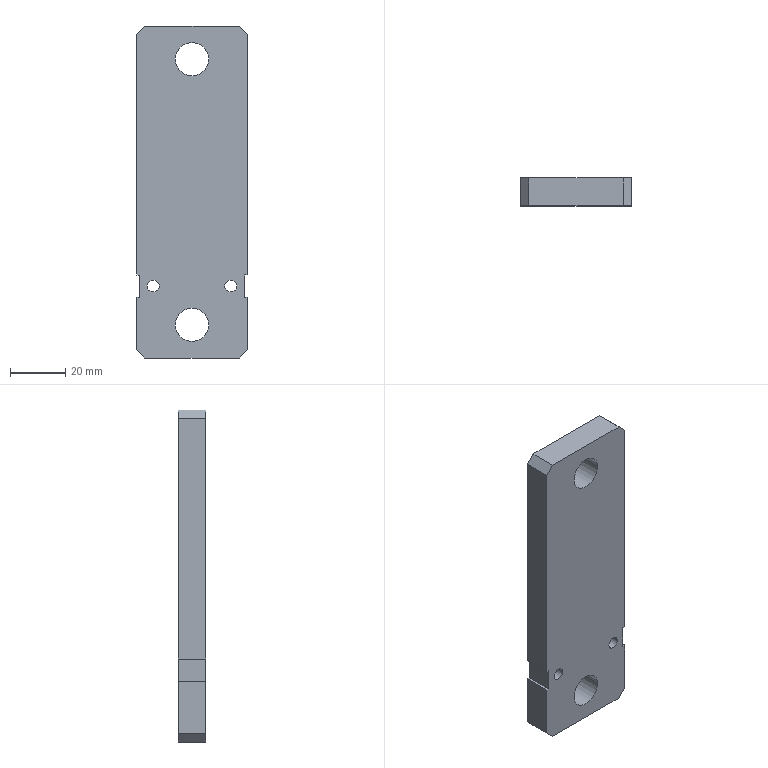Component | SolidWorks | HandlingMechanism-2_A071-1 | 1 solid | 32 faces | box 40 x 10 x 120 mm | volume 44793 mm3 | plane 20 | cylinder 12 | commonest cylinder face diameters 8 x4 4.3 x4 12 x4
build123d program:
from build123d import *

# Parameters (mm, degrees)
SKETCH4_W                                       = 40
SKETCH4_H                                       = 120
BOSS_EXTRUDE3_DEPTH                             = 10
CHAMFER1_SIZE                                   = 3
M12X1_TAPPED_HOLE1_D                            = 12
M12X1_TAPPED_HOLE1_DEPTH                        = 26.25
M12X1_TAPPED_HOLE1_TIP                          = 3.605
SKETCH8_W                                       = 1
SKETCH8_H                                       = 8
CUT_EXTRUDE2_DEPTH                              = 20
M4_HEX_SOCKET_HEAD_CAP_SCREW_CBORE1_D           = 4.3
M4_HEX_SOCKET_HEAD_CAP_SCREW_CBORE1_CBORE_D     = 8
M4_HEX_SOCKET_HEAD_CAP_SCREW_CBORE1_CBORE_DEPTH = 4.4


with BuildPart() as part:
    # Sketch4 → Boss-Extrude3 (new body)
    with BuildSketch(Plane(origin=(0, 0, 0), x_dir=(-1, 0, 0), z_dir=(0, 0, -1))):
        Rectangle(SKETCH4_W, SKETCH4_H)
    extrude(amount=BOSS_EXTRUDE3_DEPTH)

    # Chamfer1
    chamfer1_edges = [part.edges().sort_by_distance(p)[0] for p in [
        (20, 60, -5),
        (-20, 60, -5),
        (-20, -60, -5),
        (20, -60, -5),
    ]]
    chamfer(chamfer1_edges, length=CHAMFER1_SIZE)

    # M12x1 Tapped Hole1
    with Locations(Plane(origin=(0, 0, -10), x_dir=(-1, 0, 0), z_dir=(0, 0, -1))):
        with Locations((0, -48), (0, 48)):
            Hole(M12X1_TAPPED_HOLE1_D / 2, depth=M12X1_TAPPED_HOLE1_DEPTH)
            with Locations((0, 0, -(M12X1_TAPPED_HOLE1_DEPTH + M12X1_TAPPED_HOLE1_TIP / 2))):  # 118° drill point
                Cone(0, M12X1_TAPPED_HOLE1_D / 2, M12X1_TAPPED_HOLE1_TIP, mode=Mode.SUBTRACT)

    # Sketch8 → Cut-Extrude2 (cut)
    with BuildSketch(Plane(origin=(0, 0, -10), x_dir=(-1, 0, 0), z_dir=(0, 0, -1))):
        with Locations((19.5, 34)):
            Rectangle(SKETCH8_W, SKETCH8_H)
        with Locations((-19.5, 34)):
            Rectangle(SKETCH8_W, SKETCH8_H)
    extrude(amount=-CUT_EXTRUDE2_DEPTH, mode=Mode.SUBTRACT)

    # M4 Hex Socket Head Cap Screw CBORE1 (through all)
    with Locations(Plane(origin=(0, 0, -10), x_dir=(-1, 0, 0), z_dir=(0, 0, -1))):
        with Locations((-14, 34), (14, 34)):
            CounterBoreHole(M4_HEX_SOCKET_HEAD_CAP_SCREW_CBORE1_D / 2, M4_HEX_SOCKET_HEAD_CAP_SCREW_CBORE1_CBORE_D / 2, M4_HEX_SOCKET_HEAD_CAP_SCREW_CBORE1_CBORE_DEPTH)


solid = part.part

# Placed as in the assembly
solid = solid.moved(Location((25.881, 208.5, 187), (90, 0, -180)))
STEP:
#1=COLOUR_RGB('',0.7922,0.8196,0.9333);
#2=FILL_AREA_STYLE_COLOUR('',#1);
#3=FILL_AREA_STYLE('',(#2));
#4=SURFACE_STYLE_FILL_AREA(#3);
#5=SURFACE_SIDE_STYLE('',(#4));
#6=SURFACE_STYLE_USAGE(.BOTH.,#5);
#7=PRESENTATION_STYLE_ASSIGNMENT((#6));
#8=CARTESIAN_POINT('',(0.3103,8.429,6.024));
#9=VERTEX_POINT('',#8);
#10=CARTESIAN_POINT('',(0.6252,8.429,6.024));
#11=VERTEX_POINT('',#10);
#12=CARTESIAN_POINT('',(0.4677,8.429,6.024));
#13=DIRECTION('',(0.,1.,-0.));
#14=DIRECTION('',(1.,0.,0.));
#15=AXIS2_PLACEMENT_3D('',#12,#13,#14);
#16=CIRCLE('',#15,0.1575);
#17=EDGE_CURVE('',#9,#11,#16,.T.);
#18=ORIENTED_EDGE('',*,*,#17,.F.);
#19=CARTESIAN_POINT('',(0.3103,8.602,6.024));
#20=VERTEX_POINT('',#19);
#21=CARTESIAN_POINT('',(0.3103,8.602,6.024));
#22=DIRECTION('',(0.,1.,-0.));
#23=VECTOR('',#22,39.37);
#24=LINE('',#21,#23);
#25=EDGE_CURVE('',#9,#20,#24,.T.);
#26=ORIENTED_EDGE('',*,*,#25,.T.);
#27=CARTESIAN_POINT('',(0.6252,8.602,6.024));
#28=VERTEX_POINT('',#27);
#29=CARTESIAN_POINT('',(0.4677,8.602,6.024));
#30=DIRECTION('',(0.,1.,-0.));
#31=DIRECTION('',(1.,0.,0.));
#32=AXIS2_PLACEMENT_3D('',#29,#30,#31);
#33=CIRCLE('',#32,0.1575);
#34=EDGE_CURVE('',#20,#28,#33,.T.);
#35=ORIENTED_EDGE('',*,*,#34,.T.);
#36=CARTESIAN_POINT('',(0.6252,8.602,6.024));
#37=DIRECTION('',(0.,1.,-0.));
#38=VECTOR('',#37,39.37);
#39=LINE('',#36,#38);
#40=EDGE_CURVE('',#11,#28,#39,.T.);
#41=ORIENTED_EDGE('',*,*,#40,.F.);
#42=EDGE_LOOP('',(#18,#26,#35,#41));
#43=FACE_OUTER_BOUND('',#42,.T.);
#44=CARTESIAN_POINT('',(0.4677,8.602,6.024));
#45=DIRECTION('',(0.,1.,-0.));
#46=DIRECTION('',(1.,0.,0.));
#47=AXIS2_PLACEMENT_3D('',#44,#45,#46);
#48=CYLINDRICAL_SURFACE('',#47,0.1575);
#49=ADVANCED_FACE('',(#43),#48,.F.);
#50=CARTESIAN_POINT('',(0.3831,8.209,6.024));
#51=VERTEX_POINT('',#50);
#52=CARTESIAN_POINT('',(0.5524,8.209,6.024));
#53=VERTEX_POINT('',#52);
#54=CARTESIAN_POINT('',(0.4677,8.209,6.024));
#55=DIRECTION('',(0.,1.,-0.));
#56=DIRECTION('',(1.,0.,0.));
#57=AXIS2_PLACEMENT_3D('',#54,#55,#56);
#58=CIRCLE('',#57,0.08465);
#59=EDGE_CURVE('',#51,#53,#58,.T.);
#60=ORIENTED_EDGE('',*,*,#59,.F.);
#61=CARTESIAN_POINT('',(0.3831,8.429,6.024));
#62=VERTEX_POINT('',#61);
#63=CARTESIAN_POINT('',(0.3831,8.602,6.024));
#64=DIRECTION('',(0.,1.,-0.));
#65=VECTOR('',#64,39.37);
#66=LINE('',#63,#65);
#67=EDGE_CURVE('',#51,#62,#66,.T.);
#68=ORIENTED_EDGE('',*,*,#67,.T.);
#69=CARTESIAN_POINT('',(0.5524,8.429,6.024));
#70=VERTEX_POINT('',#69);
#71=CARTESIAN_POINT('',(0.4677,8.429,6.024));
#72=DIRECTION('',(0.,1.,-0.));
#73=DIRECTION('',(1.,0.,0.));
#74=AXIS2_PLACEMENT_3D('',#71,#72,#73);
#75=CIRCLE('',#74,0.08465);
#76=EDGE_CURVE('',#62,#70,#75,.T.);
#77=ORIENTED_EDGE('',*,*,#76,.T.);
#78=CARTESIAN_POINT('',(0.5524,8.602,6.024));
#79=DIRECTION('',(0.,1.,-0.));
#80=VECTOR('',#79,39.37);
#81=LINE('',#78,#80);
#82=EDGE_CURVE('',#53,#70,#81,.T.);
#83=ORIENTED_EDGE('',*,*,#82,.F.);
#84=EDGE_LOOP('',(#60,#68,#77,#83));
#85=FACE_OUTER_BOUND('',#84,.T.);
#86=CARTESIAN_POINT('',(0.4677,8.602,6.024));
#87=DIRECTION('',(0.,1.,-0.));
#88=DIRECTION('',(1.,0.,0.));
#89=AXIS2_PLACEMENT_3D('',#86,#87,#88);
#90=CYLINDRICAL_SURFACE('',#89,0.08465);
#91=ADVANCED_FACE('',(#85),#90,.F.);
#92=CARTESIAN_POINT('',(1.413,8.429,6.024));
#93=VERTEX_POINT('',#92);
#94=CARTESIAN_POINT('',(1.728,8.429,6.024));
#95=VERTEX_POINT('',#94);
#96=CARTESIAN_POINT('',(1.57,8.429,6.024));
#97=DIRECTION('',(0.,1.,-0.));
#98=DIRECTION('',(1.,0.,0.));
#99=AXIS2_PLACEMENT_3D('',#96,#97,#98);
#100=CIRCLE('',#99,0.1575);
#101=EDGE_CURVE('',#93,#95,#100,.T.);
#102=ORIENTED_EDGE('',*,*,#101,.F.);
#103=CARTESIAN_POINT('',(1.413,8.602,6.024));
#104=VERTEX_POINT('',#103);
#105=CARTESIAN_POINT('',(1.413,8.602,6.024));
#106=DIRECTION('',(0.,1.,-0.));
#107=VECTOR('',#106,39.37);
#108=LINE('',#105,#107);
#109=EDGE_CURVE('',#93,#104,#108,.T.);
#110=ORIENTED_EDGE('',*,*,#109,.T.);
#111=CARTESIAN_POINT('',(1.728,8.602,6.024));
#112=VERTEX_POINT('',#111);
#113=CARTESIAN_POINT('',(1.57,8.602,6.024));
#114=DIRECTION('',(0.,1.,-0.));
#115=DIRECTION('',(1.,0.,0.));
#116=AXIS2_PLACEMENT_3D('',#113,#114,#115);
#117=CIRCLE('',#116,0.1575);
#118=EDGE_CURVE('',#104,#112,#117,.T.);
#119=ORIENTED_EDGE('',*,*,#118,.T.);
#120=CARTESIAN_POINT('',(1.728,8.602,6.024));
#121=DIRECTION('',(0.,1.,-0.));
#122=VECTOR('',#121,39.37);
#123=LINE('',#120,#122);
#124=EDGE_CURVE('',#95,#112,#123,.T.);
#125=ORIENTED_EDGE('',*,*,#124,.F.);
#126=EDGE_LOOP('',(#102,#110,#119,#125));
#127=FACE_OUTER_BOUND('',#126,.T.);
#128=CARTESIAN_POINT('',(1.57,8.602,6.024));
#129=DIRECTION('',(0.,1.,-0.));
#130=DIRECTION('',(1.,0.,0.));
#131=AXIS2_PLACEMENT_3D('',#128,#129,#130);
#132=CYLINDRICAL_SURFACE('',#131,0.1575);
#133=ADVANCED_FACE('',(#127),#132,.F.);
#134=CARTESIAN_POINT('',(1.485,8.209,6.024));
#135=VERTEX_POINT('',#134);
#136=CARTESIAN_POINT('',(1.655,8.209,6.024));
#137=VERTEX_POINT('',#136);
#138=CARTESIAN_POINT('',(1.57,8.209,6.024));
#139=DIRECTION('',(0.,1.,-0.));
#140=DIRECTION('',(1.,0.,0.));
#141=AXIS2_PLACEMENT_3D('',#138,#139,#140);
#142=CIRCLE('',#141,0.08465);
#143=EDGE_CURVE('',#135,#137,#142,.T.);
#144=ORIENTED_EDGE('',*,*,#143,.F.);
#145=CARTESIAN_POINT('',(1.485,8.429,6.024));
#146=VERTEX_POINT('',#145);
#147=CARTESIAN_POINT('',(1.485,8.602,6.024));
#148=DIRECTION('',(0.,1.,-0.));
#149=VECTOR('',#148,39.37);
#150=LINE('',#147,#149);
#151=EDGE_CURVE('',#135,#146,#150,.T.);
#152=ORIENTED_EDGE('',*,*,#151,.T.);
#153=CARTESIAN_POINT('',(1.655,8.429,6.024));
#154=VERTEX_POINT('',#153);
#155=CARTESIAN_POINT('',(1.57,8.429,6.024));
#156=DIRECTION('',(0.,1.,-0.));
#157=DIRECTION('',(1.,0.,0.));
#158=AXIS2_PLACEMENT_3D('',#155,#156,#157);
#159=CIRCLE('',#158,0.08465);
#160=EDGE_CURVE('',#146,#154,#159,.T.);
#161=ORIENTED_EDGE('',*,*,#160,.T.);
#162=CARTESIAN_POINT('',(1.655,8.602,6.024));
#163=DIRECTION('',(0.,1.,-0.));
#164=VECTOR('',#163,39.37);
#165=LINE('',#162,#164);
#166=EDGE_CURVE('',#137,#154,#165,.T.);
#167=ORIENTED_EDGE('',*,*,#166,.F.);
#168=EDGE_LOOP('',(#144,#152,#161,#167));
#169=FACE_OUTER_BOUND('',#168,.T.);
#170=CARTESIAN_POINT('',(1.57,8.602,6.024));
#171=DIRECTION('',(0.,1.,-0.));
#172=DIRECTION('',(1.,0.,0.));
#173=AXIS2_PLACEMENT_3D('',#170,#171,#172);
#174=CYLINDRICAL_SURFACE('',#173,0.08465);
#175=ADVANCED_FACE('',(#169),#174,.F.);
#176=CARTESIAN_POINT('',(1.255,8.209,9.252));
#177=VERTEX_POINT('',#176);
#178=CARTESIAN_POINT('',(0.7827,8.209,9.252));
#179=VERTEX_POINT('',#178);
#180=CARTESIAN_POINT('',(1.019,8.209,9.252));
#181=DIRECTION('',(-0.,-1.,0.));
#182=DIRECTION('',(-1.,0.,0.));
#183=AXIS2_PLACEMENT_3D('',#180,#181,#182);
#184=CIRCLE('',#183,0.2362);
#185=EDGE_CURVE('',#177,#179,#184,.T.);
#186=ORIENTED_EDGE('',*,*,#185,.T.);
#187=CARTESIAN_POINT('',(0.7827,8.602,9.252));
#188=VERTEX_POINT('',#187);
#189=CARTESIAN_POINT('',(0.7827,8.602,9.252));
#190=DIRECTION('',(0.,1.,-0.));
#191=VECTOR('',#190,39.37);
#192=LINE('',#189,#191);
#193=EDGE_CURVE('',#179,#188,#192,.T.);
#194=ORIENTED_EDGE('',*,*,#193,.T.);
#195=CARTESIAN_POINT('',(1.255,8.602,9.252));
#196=VERTEX_POINT('',#195);
#197=CARTESIAN_POINT('',(1.019,8.602,9.252));
#198=DIRECTION('',(0.,1.,-0.));
#199=DIRECTION('',(1.,0.,0.));
#200=AXIS2_PLACEMENT_3D('',#197,#198,#199);
#201=CIRCLE('',#200,0.2362);
#202=EDGE_CURVE('',#188,#196,#201,.T.);
#203=ORIENTED_EDGE('',*,*,#202,.T.);
#204=CARTESIAN_POINT('',(1.255,8.602,9.252));
#205=DIRECTION('',(0.,1.,-0.));
#206=VECTOR('',#205,39.37);
#207=LINE('',#204,#206);
#208=EDGE_CURVE('',#177,#196,#207,.T.);
#209=ORIENTED_EDGE('',*,*,#208,.F.);
#210=EDGE_LOOP('',(#186,#194,#203,#209));
#211=FACE_OUTER_BOUND('',#210,.T.);
#212=CARTESIAN_POINT('',(1.019,8.602,9.252));
#213=DIRECTION('',(0.,1.,-0.));
#214=DIRECTION('',(1.,0.,0.));
#215=AXIS2_PLACEMENT_3D('',#212,#213,#214);
#216=CYLINDRICAL_SURFACE('',#215,0.2362);
#217=ADVANCED_FACE('',(#211),#216,.F.);
#218=CARTESIAN_POINT('',(1.255,8.209,5.472));
#219=VERTEX_POINT('',#218);
#220=CARTESIAN_POINT('',(0.7827,8.209,5.472));
#221=VERTEX_POINT('',#220);
#222=CARTESIAN_POINT('',(1.019,8.209,5.472));
#223=DIRECTION('',(-0.,-1.,0.));
#224=DIRECTION('',(-1.,0.,0.));
#225=AXIS2_PLACEMENT_3D('',#222,#223,#224);
#226=CIRCLE('',#225,0.2362);
#227=EDGE_CURVE('',#219,#221,#226,.T.);
#228=ORIENTED_EDGE('',*,*,#227,.T.);
#229=CARTESIAN_POINT('',(0.7827,8.602,5.472));
#230=VERTEX_POINT('',#229);
#231=CARTESIAN_POINT('',(0.7827,8.602,5.472));
#232=DIRECTION('',(0.,1.,-0.));
#233=VECTOR('',#232,39.37);
#234=LINE('',#231,#233);
#235=EDGE_CURVE('',#221,#230,#234,.T.);
#236=ORIENTED_EDGE('',*,*,#235,.T.);
#237=CARTESIAN_POINT('',(1.255,8.602,5.472));
#238=VERTEX_POINT('',#237);
#239=CARTESIAN_POINT('',(1.019,8.602,5.472));
#240=DIRECTION('',(0.,1.,-0.));
#241=DIRECTION('',(1.,0.,0.));
#242=AXIS2_PLACEMENT_3D('',#239,#240,#241);
#243=CIRCLE('',#242,0.2362);
#244=EDGE_CURVE('',#230,#238,#243,.T.);
#245=ORIENTED_EDGE('',*,*,#244,.T.);
#246=CARTESIAN_POINT('',(1.255,8.602,5.472));
#247=DIRECTION('',(0.,1.,-0.));
#248=VECTOR('',#247,39.37);
#249=LINE('',#246,#248);
#250=EDGE_CURVE('',#219,#238,#249,.T.);
#251=ORIENTED_EDGE('',*,*,#250,.F.);
#252=EDGE_LOOP('',(#228,#236,#245,#251));
#253=FACE_OUTER_BOUND('',#252,.T.);
#254=CARTESIAN_POINT('',(1.019,8.602,5.472));
#255=DIRECTION('',(0.,1.,-0.));
#256=DIRECTION('',(1.,0.,0.));
#257=AXIS2_PLACEMENT_3D('',#254,#255,#256);
#258=CYLINDRICAL_SURFACE('',#257,0.2362);
#259=ADVANCED_FACE('',(#253),#258,.F.);
#260=CARTESIAN_POINT('',(1.57,8.602,6.024));
#261=DIRECTION('',(0.,1.,-0.));
#262=DIRECTION('',(1.,0.,0.));
#263=AXIS2_PLACEMENT_3D('',#260,#261,#262);
#264=CIRCLE('',#263,0.1575);
#265=EDGE_CURVE('',#112,#104,#264,.T.);
#266=ORIENTED_EDGE('',*,*,#265,.F.);
#267=ORIENTED_EDGE('',*,*,#118,.F.);
#268=EDGE_LOOP('',(#266,#267));
#269=FACE_BOUND('',#268,.T.);
#270=CARTESIAN_POINT('',(1.019,8.602,9.252));
#271=DIRECTION('',(0.,1.,-0.));
#272=DIRECTION('',(1.,0.,0.));
#273=AXIS2_PLACEMENT_3D('',#270,#271,#272);
#274=CIRCLE('',#273,0.2362);
#275=EDGE_CURVE('',#196,#188,#274,.T.);
#276=ORIENTED_EDGE('',*,*,#275,.F.);
#277=ORIENTED_EDGE('',*,*,#202,.F.);
#278=EDGE_LOOP('',(#276,#277));
#279=FACE_BOUND('',#278,.T.);
#280=CARTESIAN_POINT('',(1.019,8.602,5.472));
#281=DIRECTION('',(0.,1.,-0.));
#282=DIRECTION('',(1.,0.,0.));
#283=AXIS2_PLACEMENT_3D('',#280,#281,#282);
#284=CIRCLE('',#283,0.2362);
#285=EDGE_CURVE('',#238,#230,#284,.T.);
#286=ORIENTED_EDGE('',*,*,#285,.F.);
#287=ORIENTED_EDGE('',*,*,#244,.F.);
#288=EDGE_LOOP('',(#286,#287));
#289=FACE_BOUND('',#288,.T.);
#290=CARTESIAN_POINT('',(0.2709,8.602,6.181));
#291=VERTEX_POINT('',#290);
#292=CARTESIAN_POINT('',(0.2709,8.602,5.866));
#293=VERTEX_POINT('',#292);
#294=CARTESIAN_POINT('',(0.2709,8.602,5.866));
#295=DIRECTION('',(0.,-0.,-1.));
#296=VECTOR('',#295,39.37);
#297=LINE('',#294,#296);
#298=EDGE_CURVE('',#291,#293,#297,.T.);
#299=ORIENTED_EDGE('',*,*,#298,.F.);
#300=CARTESIAN_POINT('',(0.2315,8.602,6.181));
#301=VERTEX_POINT('',#300);
#302=CARTESIAN_POINT('',(0.2709,8.602,6.181));
#303=DIRECTION('',(1.,-0.,0.));
#304=VECTOR('',#303,39.37);
#305=LINE('',#302,#304);
#306=EDGE_CURVE('',#301,#291,#305,.T.);
#307=ORIENTED_EDGE('',*,*,#306,.F.);
#308=CARTESIAN_POINT('',(0.2315,8.602,9.606));
#309=VERTEX_POINT('',#308);
#310=CARTESIAN_POINT('',(0.2315,8.602,9.724));
#311=DIRECTION('',(-0.,0.,1.));
#312=VECTOR('',#311,39.37);
#313=LINE('',#310,#312);
#314=EDGE_CURVE('',#301,#309,#313,.T.);
#315=ORIENTED_EDGE('',*,*,#314,.T.);
#316=CARTESIAN_POINT('',(0.3496,8.602,9.724));
#317=VERTEX_POINT('',#316);
#318=CARTESIAN_POINT('',(0.3496,8.602,9.724));
#319=DIRECTION('',(0.7071,-0.,0.7071));
#320=VECTOR('',#319,39.37);
#321=LINE('',#318,#320);
#322=EDGE_CURVE('',#309,#317,#321,.T.);
#323=ORIENTED_EDGE('',*,*,#322,.T.);
#324=CARTESIAN_POINT('',(1.688,8.602,9.724));
#325=VERTEX_POINT('',#324);
#326=CARTESIAN_POINT('',(0.2315,8.602,9.724));
#327=DIRECTION('',(1.,-0.,0.));
#328=VECTOR('',#327,39.37);
#329=LINE('',#326,#328);
#330=EDGE_CURVE('',#317,#325,#329,.T.);
#331=ORIENTED_EDGE('',*,*,#330,.T.);
#332=CARTESIAN_POINT('',(1.806,8.602,9.606));
#333=VERTEX_POINT('',#332);
#334=CARTESIAN_POINT('',(1.806,8.602,9.606));
#335=DIRECTION('',(0.7071,-0.,-0.7071));
#336=VECTOR('',#335,39.37);
#337=LINE('',#334,#336);
#338=EDGE_CURVE('',#325,#333,#337,.T.);
#339=ORIENTED_EDGE('',*,*,#338,.T.);
#340=CARTESIAN_POINT('',(1.806,8.602,6.181));
#341=VERTEX_POINT('',#340);
#342=CARTESIAN_POINT('',(1.806,8.602,9.724));
#343=DIRECTION('',(0.,-0.,-1.));
#344=VECTOR('',#343,39.37);
#345=LINE('',#342,#344);
#346=EDGE_CURVE('',#333,#341,#345,.T.);
#347=ORIENTED_EDGE('',*,*,#346,.T.);
#348=CARTESIAN_POINT('',(1.767,8.602,6.181));
#349=VERTEX_POINT('',#348);
#350=CARTESIAN_POINT('',(1.767,8.602,6.181));
#351=DIRECTION('',(1.,-0.,0.));
#352=VECTOR('',#351,39.37);
#353=LINE('',#350,#352);
#354=EDGE_CURVE('',#349,#341,#353,.T.);
#355=ORIENTED_EDGE('',*,*,#354,.F.);
#356=CARTESIAN_POINT('',(1.767,8.602,5.866));
#357=VERTEX_POINT('',#356);
#358=CARTESIAN_POINT('',(1.767,8.602,5.866));
#359=DIRECTION('',(-0.,0.,1.));
#360=VECTOR('',#359,39.37);
#361=LINE('',#358,#360);
#362=EDGE_CURVE('',#357,#349,#361,.T.);
#363=ORIENTED_EDGE('',*,*,#362,.F.);
#364=CARTESIAN_POINT('',(1.806,8.602,5.866));
#365=VERTEX_POINT('',#364);
#366=CARTESIAN_POINT('',(1.767,8.602,5.866));
#367=DIRECTION('',(-1.,0.,-0.));
#368=VECTOR('',#367,39.37);
#369=LINE('',#366,#368);
#370=EDGE_CURVE('',#365,#357,#369,.T.);
#371=ORIENTED_EDGE('',*,*,#370,.F.);
#372=CARTESIAN_POINT('',(1.806,8.602,5.118));
#373=VERTEX_POINT('',#372);
#374=CARTESIAN_POINT('',(1.806,8.602,9.724));
#375=DIRECTION('',(0.,-0.,-1.));
#376=VECTOR('',#375,39.37);
#377=LINE('',#374,#376);
#378=EDGE_CURVE('',#365,#373,#377,.T.);
#379=ORIENTED_EDGE('',*,*,#378,.T.);
#380=CARTESIAN_POINT('',(1.688,8.602,5.));
#381=VERTEX_POINT('',#380);
#382=CARTESIAN_POINT('',(1.688,8.602,5.));
#383=DIRECTION('',(-0.7071,0.,-0.7071));
#384=VECTOR('',#383,39.37);
#385=LINE('',#382,#384);
#386=EDGE_CURVE('',#373,#381,#385,.T.);
#387=ORIENTED_EDGE('',*,*,#386,.T.);
#388=CARTESIAN_POINT('',(0.3496,8.602,5.));
#389=VERTEX_POINT('',#388);
#390=CARTESIAN_POINT('',(0.2315,8.602,5.));
#391=DIRECTION('',(-1.,0.,-0.));
#392=VECTOR('',#391,39.37);
#393=LINE('',#390,#392);
#394=EDGE_CURVE('',#381,#389,#393,.T.);
#395=ORIENTED_EDGE('',*,*,#394,.T.);
#396=CARTESIAN_POINT('',(0.2315,8.602,5.118));
#397=VERTEX_POINT('',#396);
#398=CARTESIAN_POINT('',(0.2315,8.602,5.118));
#399=DIRECTION('',(-0.7071,0.,0.7071));
#400=VECTOR('',#399,39.37);
#401=LINE('',#398,#400);
#402=EDGE_CURVE('',#389,#397,#401,.T.);
#403=ORIENTED_EDGE('',*,*,#402,.T.);
#404=CARTESIAN_POINT('',(0.2315,8.602,5.866));
#405=VERTEX_POINT('',#404);
#406=CARTESIAN_POINT('',(0.2315,8.602,9.724));
#407=DIRECTION('',(-0.,0.,1.));
#408=VECTOR('',#407,39.37);
#409=LINE('',#406,#408);
#410=EDGE_CURVE('',#397,#405,#409,.T.);
#411=ORIENTED_EDGE('',*,*,#410,.T.);
#412=CARTESIAN_POINT('',(0.2709,8.602,5.866));
#413=DIRECTION('',(-1.,0.,-0.));
#414=VECTOR('',#413,39.37);
#415=LINE('',#412,#414);
#416=EDGE_CURVE('',#293,#405,#415,.T.);
#417=ORIENTED_EDGE('',*,*,#416,.F.);
#418=EDGE_LOOP('',(#299,#307,#315,#323,#331,#339,#347,#355,#363,#371,#379,#387,#395,#403,#411,#417));
#419=FACE_OUTER_BOUND('',#418,.T.);
#420=CARTESIAN_POINT('',(0.4677,8.602,6.024));
#421=DIRECTION('',(0.,1.,-0.));
#422=DIRECTION('',(1.,0.,0.));
#423=AXIS2_PLACEMENT_3D('',#420,#421,#422);
#424=CIRCLE('',#423,0.1575);
#425=EDGE_CURVE('',#28,#20,#424,.T.);
#426=ORIENTED_EDGE('',*,*,#425,.F.);
#427=ORIENTED_EDGE('',*,*,#34,.F.);
#428=EDGE_LOOP('',(#426,#427));
#429=FACE_BOUND('',#428,.T.);
#430=CARTESIAN_POINT('',(1.019,8.602,7.362));
#431=DIRECTION('',(-0.,-1.,0.));
#432=DIRECTION('',(-1.,0.,-0.));
#433=AXIS2_PLACEMENT_3D('',#430,#431,#432);
#434=PLANE('',#433);
#435=ADVANCED_FACE('',(#269,#279,#289,#419,#429),#434,.F.);
#436=ORIENTED_EDGE('',*,*,#314,.F.);
#437=CARTESIAN_POINT('',(0.2315,8.209,6.181));
#438=VERTEX_POINT('',#437);
#439=CARTESIAN_POINT('',(0.2315,7.815,6.181));
#440=DIRECTION('',(0.,1.,-0.));
#441=VECTOR('',#440,39.37);
#442=LINE('',#439,#441);
#443=EDGE_CURVE('',#438,#301,#442,.T.);
#444=ORIENTED_EDGE('',*,*,#443,.F.);
#445=CARTESIAN_POINT('',(0.2315,8.209,9.606));
#446=VERTEX_POINT('',#445);
#447=CARTESIAN_POINT('',(0.2315,8.209,9.724));
#448=DIRECTION('',(-0.,0.,1.));
#449=VECTOR('',#448,39.37);
#450=LINE('',#447,#449);
#451=EDGE_CURVE('',#438,#446,#450,.T.);
#452=ORIENTED_EDGE('',*,*,#451,.T.);
#453=CARTESIAN_POINT('',(0.2315,8.602,9.606));
#454=DIRECTION('',(0.,1.,-0.));
#455=VECTOR('',#454,39.37);
#456=LINE('',#453,#455);
#457=EDGE_CURVE('',#446,#309,#456,.T.);
#458=ORIENTED_EDGE('',*,*,#457,.T.);
#459=EDGE_LOOP('',(#436,#444,#452,#458));
#460=FACE_OUTER_BOUND('',#459,.T.);
#461=CARTESIAN_POINT('',(0.2315,8.602,9.724));
#462=DIRECTION('',(1.,-0.,0.));
#463=DIRECTION('',(-0.,-1.,0.));
#464=AXIS2_PLACEMENT_3D('',#461,#462,#463);
#465=PLANE('',#464);
#466=ADVANCED_FACE('',(#460),#465,.F.);
#467=ORIENTED_EDGE('',*,*,#378,.F.);
#468=CARTESIAN_POINT('',(1.806,8.209,5.866));
#469=VERTEX_POINT('',#468);
#470=CARTESIAN_POINT('',(1.806,7.815,5.866));
#471=DIRECTION('',(0.,1.,-0.));
#472=VECTOR('',#471,39.37);
#473=LINE('',#470,#472);
#474=EDGE_CURVE('',#469,#365,#473,.T.);
#475=ORIENTED_EDGE('',*,*,#474,.F.);
#476=CARTESIAN_POINT('',(1.806,8.209,5.118));
#477=VERTEX_POINT('',#476);
#478=CARTESIAN_POINT('',(1.806,8.209,9.724));
#479=DIRECTION('',(0.,-0.,-1.));
#480=VECTOR('',#479,39.37);
#481=LINE('',#478,#480);
#482=EDGE_CURVE('',#469,#477,#481,.T.);
#483=ORIENTED_EDGE('',*,*,#482,.T.);
#484=CARTESIAN_POINT('',(1.806,8.602,5.118));
#485=DIRECTION('',(0.,1.,-0.));
#486=VECTOR('',#485,39.37);
#487=LINE('',#484,#486);
#488=EDGE_CURVE('',#477,#373,#487,.T.);
#489=ORIENTED_EDGE('',*,*,#488,.T.);
#490=EDGE_LOOP('',(#467,#475,#483,#489));
#491=FACE_OUTER_BOUND('',#490,.T.);
#492=CARTESIAN_POINT('',(1.806,8.602,9.724));
#493=DIRECTION('',(-1.,0.,-0.));
#494=DIRECTION('',(0.,1.,-0.));
#495=AXIS2_PLACEMENT_3D('',#492,#493,#494);
#496=PLANE('',#495);
#497=ADVANCED_FACE('',(#491),#496,.F.);
#498=CARTESIAN_POINT('',(0.2315,8.209,5.118));
#499=VERTEX_POINT('',#498);
#500=CARTESIAN_POINT('',(0.2315,8.209,5.866));
#501=VERTEX_POINT('',#500);
#502=CARTESIAN_POINT('',(0.2315,8.209,9.724));
#503=DIRECTION('',(-0.,0.,1.));
#504=VECTOR('',#503,39.37);
#505=LINE('',#502,#504);
#506=EDGE_CURVE('',#499,#501,#505,.T.);
#507=ORIENTED_EDGE('',*,*,#506,.T.);
#508=CARTESIAN_POINT('',(0.2315,7.815,5.866));
#509=DIRECTION('',(0.,1.,-0.));
#510=VECTOR('',#509,39.37);
#511=LINE('',#508,#510);
#512=EDGE_CURVE('',#501,#405,#511,.T.);
#513=ORIENTED_EDGE('',*,*,#512,.T.);
#514=ORIENTED_EDGE('',*,*,#410,.F.);
#515=CARTESIAN_POINT('',(0.2315,8.602,5.118));
#516=DIRECTION('',(-0.,-1.,0.));
#517=VECTOR('',#516,39.37);
#518=LINE('',#515,#517);
#519=EDGE_CURVE('',#397,#499,#518,.T.);
#520=ORIENTED_EDGE('',*,*,#519,.T.);
#521=EDGE_LOOP('',(#507,#513,#514,#520));
#522=FACE_OUTER_BOUND('',#521,.T.);
#523=CARTESIAN_POINT('',(0.2315,8.602,9.724));
#524=DIRECTION('',(1.,-0.,0.));
#525=DIRECTION('',(-0.,-1.,0.));
#526=AXIS2_PLACEMENT_3D('',#523,#524,#525);
#527=PLANE('',#526);
#528=ADVANCED_FACE('',(#522),#527,.F.);
#529=CARTESIAN_POINT('',(0.3496,8.209,9.724));
#530=VERTEX_POINT('',#529);
#531=CARTESIAN_POINT('',(1.688,8.209,9.724));
#532=VERTEX_POINT('',#531);
#533=CARTESIAN_POINT('',(0.2315,8.209,9.724));
#534=DIRECTION('',(1.,-0.,0.));
#535=VECTOR('',#534,39.37);
#536=LINE('',#533,#535);
#537=EDGE_CURVE('',#530,#532,#536,.T.);
#538=ORIENTED_EDGE('',*,*,#537,.T.);
#539=CARTESIAN_POINT('',(1.688,8.602,9.724));
#540=DIRECTION('',(0.,1.,-0.));
#541=VECTOR('',#540,39.37);
#542=LINE('',#539,#541);
#543=EDGE_CURVE('',#532,#325,#542,.T.);
#544=ORIENTED_EDGE('',*,*,#543,.T.);
#545=ORIENTED_EDGE('',*,*,#330,.F.);
#546=CARTESIAN_POINT('',(0.3496,8.602,9.724));
#547=DIRECTION('',(-0.,-1.,0.));
#548=VECTOR('',#547,39.37);
#549=LINE('',#546,#548);
#550=EDGE_CURVE('',#317,#530,#549,.T.);
#551=ORIENTED_EDGE('',*,*,#550,.T.);
#552=EDGE_LOOP('',(#538,#544,#545,#551));
#553=FACE_OUTER_BOUND('',#552,.T.);
#554=CARTESIAN_POINT('',(0.2315,8.602,9.724));
#555=DIRECTION('',(0.,-0.,-1.));
#556=DIRECTION('',(-0.,-1.,0.));
#557=AXIS2_PLACEMENT_3D('',#554,#555,#556);
#558=PLANE('',#557);
#559=ADVANCED_FACE('',(#553),#558,.F.);
#560=CARTESIAN_POINT('',(1.806,8.209,9.606));
#561=VERTEX_POINT('',#560);
#562=CARTESIAN_POINT('',(1.806,8.209,6.181));
#563=VERTEX_POINT('',#562);
#564=CARTESIAN_POINT('',(1.806,8.209,9.724));
#565=DIRECTION('',(0.,-0.,-1.));
#566=VECTOR('',#565,39.37);
#567=LINE('',#564,#566);
#568=EDGE_CURVE('',#561,#563,#567,.T.);
#569=ORIENTED_EDGE('',*,*,#568,.T.);
#570=CARTESIAN_POINT('',(1.806,7.815,6.181));
#571=DIRECTION('',(0.,1.,-0.));
#572=VECTOR('',#571,39.37);
#573=LINE('',#570,#572);
#574=EDGE_CURVE('',#563,#341,#573,.T.);
#575=ORIENTED_EDGE('',*,*,#574,.T.);
#576=ORIENTED_EDGE('',*,*,#346,.F.);
#577=CARTESIAN_POINT('',(1.806,8.602,9.606));
#578=DIRECTION('',(-0.,-1.,0.));
#579=VECTOR('',#578,39.37);
#580=LINE('',#577,#579);
#581=EDGE_CURVE('',#333,#561,#580,.T.);
#582=ORIENTED_EDGE('',*,*,#581,.T.);
#583=EDGE_LOOP('',(#569,#575,#576,#582));
#584=FACE_OUTER_BOUND('',#583,.T.);
#585=CARTESIAN_POINT('',(1.806,8.602,9.724));
#586=DIRECTION('',(-1.,0.,-0.));
#587=DIRECTION('',(0.,1.,-0.));
#588=AXIS2_PLACEMENT_3D('',#585,#586,#587);
#589=PLANE('',#588);
#590=ADVANCED_FACE('',(#584),#589,.F.);
#591=ORIENTED_EDGE('',*,*,#394,.F.);
#592=CARTESIAN_POINT('',(1.688,8.209,5.));
#593=VERTEX_POINT('',#592);
#594=CARTESIAN_POINT('',(1.688,8.602,5.));
#595=DIRECTION('',(-0.,-1.,0.));
#596=VECTOR('',#595,39.37);
#597=LINE('',#594,#596);
#598=EDGE_CURVE('',#381,#593,#597,.T.);
#599=ORIENTED_EDGE('',*,*,#598,.T.);
#600=CARTESIAN_POINT('',(0.3496,8.209,5.));
#601=VERTEX_POINT('',#600);
#602=CARTESIAN_POINT('',(0.2315,8.209,5.));
#603=DIRECTION('',(-1.,0.,-0.));
#604=VECTOR('',#603,39.37);
#605=LINE('',#602,#604);
#606=EDGE_CURVE('',#593,#601,#605,.T.);
#607=ORIENTED_EDGE('',*,*,#606,.T.);
#608=CARTESIAN_POINT('',(0.3496,8.602,5.));
#609=DIRECTION('',(0.,1.,-0.));
#610=VECTOR('',#609,39.37);
#611=LINE('',#608,#610);
#612=EDGE_CURVE('',#601,#389,#611,.T.);
#613=ORIENTED_EDGE('',*,*,#612,.T.);
#614=EDGE_LOOP('',(#591,#599,#607,#613));
#615=FACE_OUTER_BOUND('',#614,.T.);
#616=CARTESIAN_POINT('',(0.2315,8.602,5.));
#617=DIRECTION('',(-0.,0.,1.));
#618=DIRECTION('',(-1.,0.,-0.));
#619=AXIS2_PLACEMENT_3D('',#616,#617,#618);
#620=PLANE('',#619);
#621=ADVANCED_FACE('',(#615),#620,.F.);
#622=CARTESIAN_POINT('',(0.4677,8.209,6.024));
#623=DIRECTION('',(0.,1.,-0.));
#624=DIRECTION('',(1.,0.,0.));
#625=AXIS2_PLACEMENT_3D('',#622,#623,#624);
#626=CIRCLE('',#625,0.08465);
#627=EDGE_CURVE('',#53,#51,#626,.T.);
#628=ORIENTED_EDGE('',*,*,#627,.T.);
#629=ORIENTED_EDGE('',*,*,#59,.T.);
#630=EDGE_LOOP('',(#628,#629));
#631=FACE_BOUND('',#630,.T.);
#632=CARTESIAN_POINT('',(1.57,8.209,6.024));
#633=DIRECTION('',(0.,1.,-0.));
#634=DIRECTION('',(1.,0.,0.));
#635=AXIS2_PLACEMENT_3D('',#632,#633,#634);
#636=CIRCLE('',#635,0.08465);
#637=EDGE_CURVE('',#137,#135,#636,.T.);
#638=ORIENTED_EDGE('',*,*,#637,.T.);
#639=ORIENTED_EDGE('',*,*,#143,.T.);
#640=EDGE_LOOP('',(#638,#639));
#641=FACE_BOUND('',#640,.T.);
#642=CARTESIAN_POINT('',(0.2709,8.209,6.181));
#643=VERTEX_POINT('',#642);
#644=CARTESIAN_POINT('',(1.019,8.209,6.181));
#645=DIRECTION('',(-1.,0.,-0.));
#646=VECTOR('',#645,39.37);
#647=LINE('',#644,#646);
#648=EDGE_CURVE('',#643,#438,#647,.T.);
#649=ORIENTED_EDGE('',*,*,#648,.F.);
#650=CARTESIAN_POINT('',(0.2709,8.209,5.866));
#651=VERTEX_POINT('',#650);
#652=CARTESIAN_POINT('',(0.2709,8.209,7.362));
#653=DIRECTION('',(-0.,0.,1.));
#654=VECTOR('',#653,39.37);
#655=LINE('',#652,#654);
#656=EDGE_CURVE('',#651,#643,#655,.T.);
#657=ORIENTED_EDGE('',*,*,#656,.F.);
#658=CARTESIAN_POINT('',(1.019,8.209,5.866));
#659=DIRECTION('',(1.,-0.,0.));
#660=VECTOR('',#659,39.37);
#661=LINE('',#658,#660);
#662=EDGE_CURVE('',#501,#651,#661,.T.);
#663=ORIENTED_EDGE('',*,*,#662,.F.);
#664=ORIENTED_EDGE('',*,*,#506,.F.);
#665=CARTESIAN_POINT('',(-0.4968,8.209,5.846));
#666=DIRECTION('',(0.7071,-0.,-0.7071));
#667=VECTOR('',#666,39.37);
#668=LINE('',#665,#667);
#669=EDGE_CURVE('',#499,#601,#668,.T.);
#670=ORIENTED_EDGE('',*,*,#669,.T.);
#671=ORIENTED_EDGE('',*,*,#606,.F.);
#672=CARTESIAN_POINT('',(2.535,8.209,5.846));
#673=DIRECTION('',(0.7071,-0.,0.7071));
#674=VECTOR('',#673,39.37);
#675=LINE('',#672,#674);
#676=EDGE_CURVE('',#593,#477,#675,.T.);
#677=ORIENTED_EDGE('',*,*,#676,.T.);
#678=ORIENTED_EDGE('',*,*,#482,.F.);
#679=CARTESIAN_POINT('',(1.767,8.209,5.866));
#680=VERTEX_POINT('',#679);
#681=CARTESIAN_POINT('',(1.019,8.209,5.866));
#682=DIRECTION('',(1.,-0.,0.));
#683=VECTOR('',#682,39.37);
#684=LINE('',#681,#683);
#685=EDGE_CURVE('',#680,#469,#684,.T.);
#686=ORIENTED_EDGE('',*,*,#685,.F.);
#687=CARTESIAN_POINT('',(1.767,8.209,6.181));
#688=VERTEX_POINT('',#687);
#689=CARTESIAN_POINT('',(1.767,8.209,7.362));
#690=DIRECTION('',(0.,-0.,-1.));
#691=VECTOR('',#690,39.37);
#692=LINE('',#689,#691);
#693=EDGE_CURVE('',#688,#680,#692,.T.);
#694=ORIENTED_EDGE('',*,*,#693,.F.);
#695=CARTESIAN_POINT('',(1.019,8.209,6.181));
#696=DIRECTION('',(-1.,0.,-0.));
#697=VECTOR('',#696,39.37);
#698=LINE('',#695,#697);
#699=EDGE_CURVE('',#563,#688,#698,.T.);
#700=ORIENTED_EDGE('',*,*,#699,.F.);
#701=ORIENTED_EDGE('',*,*,#568,.F.);
#702=CARTESIAN_POINT('',(2.535,8.209,8.878));
#703=DIRECTION('',(-0.7071,0.,0.7071));
#704=VECTOR('',#703,39.37);
#705=LINE('',#702,#704);
#706=EDGE_CURVE('',#561,#532,#705,.T.);
#707=ORIENTED_EDGE('',*,*,#706,.T.);
#708=ORIENTED_EDGE('',*,*,#537,.F.);
#709=CARTESIAN_POINT('',(-0.4968,8.209,8.878));
#710=DIRECTION('',(-0.7071,0.,-0.7071));
#711=VECTOR('',#710,39.37);
#712=LINE('',#709,#711);
#713=EDGE_CURVE('',#530,#446,#712,.T.);
#714=ORIENTED_EDGE('',*,*,#713,.T.);
#715=ORIENTED_EDGE('',*,*,#451,.F.);
#716=EDGE_LOOP('',(#649,#657,#663,#664,#670,#671,#677,#678,#686,#694,#700,#701,#707,#708,#714,#715));
#717=FACE_OUTER_BOUND('',#716,.T.);
#718=ORIENTED_EDGE('',*,*,#185,.F.);
#719=CARTESIAN_POINT('',(1.019,8.209,9.252));
#720=DIRECTION('',(-0.,-1.,0.));
#721=DIRECTION('',(-1.,0.,0.));
#722=AXIS2_PLACEMENT_3D('',#719,#720,#721);
#723=CIRCLE('',#722,0.2362);
#724=EDGE_CURVE('',#179,#177,#723,.T.);
#725=ORIENTED_EDGE('',*,*,#724,.F.);
#726=EDGE_LOOP('',(#718,#725));
#727=FACE_BOUND('',#726,.T.);
#728=ORIENTED_EDGE('',*,*,#227,.F.);
#729=CARTESIAN_POINT('',(1.019,8.209,5.472));
#730=DIRECTION('',(-0.,-1.,0.));
#731=DIRECTION('',(-1.,0.,0.));
#732=AXIS2_PLACEMENT_3D('',#729,#730,#731);
#733=CIRCLE('',#732,0.2362);
#734=EDGE_CURVE('',#221,#219,#733,.T.);
#735=ORIENTED_EDGE('',*,*,#734,.F.);
#736=EDGE_LOOP('',(#728,#735));
#737=FACE_BOUND('',#736,.T.);
#738=CARTESIAN_POINT('',(1.019,8.209,7.362));
#739=DIRECTION('',(-0.,-1.,0.));
#740=DIRECTION('',(-1.,0.,-0.));
#741=AXIS2_PLACEMENT_3D('',#738,#739,#740);
#742=PLANE('',#741);
#743=ADVANCED_FACE('',(#631,#641,#717,#727,#737),#742,.T.);
#744=ORIENTED_EDGE('',*,*,#386,.F.);
#745=ORIENTED_EDGE('',*,*,#488,.F.);
#746=ORIENTED_EDGE('',*,*,#676,.F.);
#747=ORIENTED_EDGE('',*,*,#598,.F.);
#748=EDGE_LOOP('',(#744,#745,#746,#747));
#749=FACE_OUTER_BOUND('',#748,.T.);
#750=CARTESIAN_POINT('',(1.688,8.602,5.));
#751=DIRECTION('',(-0.7071,0.,0.7071));
#752=DIRECTION('',(-0.,-1.,0.));
#753=AXIS2_PLACEMENT_3D('',#750,#751,#752);
#754=PLANE('',#753);
#755=ADVANCED_FACE('',(#749),#754,.F.);
#756=ORIENTED_EDGE('',*,*,#402,.F.);
#757=ORIENTED_EDGE('',*,*,#612,.F.);
#758=ORIENTED_EDGE('',*,*,#669,.F.);
#759=ORIENTED_EDGE('',*,*,#519,.F.);
#760=EDGE_LOOP('',(#756,#757,#758,#759));
#761=FACE_OUTER_BOUND('',#760,.T.);
#762=CARTESIAN_POINT('',(0.2315,8.602,5.118));
#763=DIRECTION('',(0.7071,0.,0.7071));
#764=DIRECTION('',(-0.,-1.,0.));
#765=AXIS2_PLACEMENT_3D('',#762,#763,#764);
#766=PLANE('',#765);
#767=ADVANCED_FACE('',(#761),#766,.F.);
#768=ORIENTED_EDGE('',*,*,#338,.F.);
#769=ORIENTED_EDGE('',*,*,#543,.F.);
#770=ORIENTED_EDGE('',*,*,#706,.F.);
#771=ORIENTED_EDGE('',*,*,#581,.F.);
#772=EDGE_LOOP('',(#768,#769,#770,#771));
#773=FACE_OUTER_BOUND('',#772,.T.);
#774=CARTESIAN_POINT('',(1.806,8.602,9.606));
#775=DIRECTION('',(-0.7071,-0.,-0.7071));
#776=DIRECTION('',(-0.,-1.,0.));
#777=AXIS2_PLACEMENT_3D('',#774,#775,#776);
#778=PLANE('',#777);
#779=ADVANCED_FACE('',(#773),#778,.F.);
#780=ORIENTED_EDGE('',*,*,#322,.F.);
#781=ORIENTED_EDGE('',*,*,#457,.F.);
#782=ORIENTED_EDGE('',*,*,#713,.F.);
#783=ORIENTED_EDGE('',*,*,#550,.F.);
#784=EDGE_LOOP('',(#780,#781,#782,#783));
#785=FACE_OUTER_BOUND('',#784,.T.);
#786=CARTESIAN_POINT('',(0.3496,8.602,9.724));
#787=DIRECTION('',(0.7071,-0.,-0.7071));
#788=DIRECTION('',(-0.,-1.,0.));
#789=AXIS2_PLACEMENT_3D('',#786,#787,#788);
#790=PLANE('',#789);
#791=ADVANCED_FACE('',(#785),#790,.F.);
#792=ORIENTED_EDGE('',*,*,#235,.F.);
#793=ORIENTED_EDGE('',*,*,#734,.T.);
#794=ORIENTED_EDGE('',*,*,#250,.T.);
#795=ORIENTED_EDGE('',*,*,#285,.T.);
#796=EDGE_LOOP('',(#792,#793,#794,#795));
#797=FACE_OUTER_BOUND('',#796,.T.);
#798=CARTESIAN_POINT('',(1.019,8.602,5.472));
#799=DIRECTION('',(0.,1.,-0.));
#800=DIRECTION('',(1.,0.,0.));
#801=AXIS2_PLACEMENT_3D('',#798,#799,#800);
#802=CYLINDRICAL_SURFACE('',#801,0.2362);
#803=ADVANCED_FACE('',(#797),#802,.F.);
#804=ORIENTED_EDGE('',*,*,#193,.F.);
#805=ORIENTED_EDGE('',*,*,#724,.T.);
#806=ORIENTED_EDGE('',*,*,#208,.T.);
#807=ORIENTED_EDGE('',*,*,#275,.T.);
#808=EDGE_LOOP('',(#804,#805,#806,#807));
#809=FACE_OUTER_BOUND('',#808,.T.);
#810=CARTESIAN_POINT('',(1.019,8.602,9.252));
#811=DIRECTION('',(0.,1.,-0.));
#812=DIRECTION('',(1.,0.,0.));
#813=AXIS2_PLACEMENT_3D('',#810,#811,#812);
#814=CYLINDRICAL_SURFACE('',#813,0.2362);
#815=ADVANCED_FACE('',(#809),#814,.F.);
#816=ORIENTED_EDGE('',*,*,#693,.T.);
#817=CARTESIAN_POINT('',(1.767,7.815,5.866));
#818=DIRECTION('',(0.,1.,-0.));
#819=VECTOR('',#818,39.37);
#820=LINE('',#817,#819);
#821=EDGE_CURVE('',#680,#357,#820,.T.);
#822=ORIENTED_EDGE('',*,*,#821,.T.);
#823=ORIENTED_EDGE('',*,*,#362,.T.);
#824=CARTESIAN_POINT('',(1.767,7.815,6.181));
#825=DIRECTION('',(0.,1.,-0.));
#826=VECTOR('',#825,39.37);
#827=LINE('',#824,#826);
#828=EDGE_CURVE('',#688,#349,#827,.T.);
#829=ORIENTED_EDGE('',*,*,#828,.F.);
#830=EDGE_LOOP('',(#816,#822,#823,#829));
#831=FACE_OUTER_BOUND('',#830,.T.);
#832=CARTESIAN_POINT('',(1.767,7.815,5.866));
#833=DIRECTION('',(-1.,0.,-0.));
#834=DIRECTION('',(0.,1.,-0.));
#835=AXIS2_PLACEMENT_3D('',#832,#833,#834);
#836=PLANE('',#835);
#837=ADVANCED_FACE('',(#831),#836,.F.);
#838=ORIENTED_EDGE('',*,*,#685,.T.);
#839=ORIENTED_EDGE('',*,*,#474,.T.);
#840=ORIENTED_EDGE('',*,*,#370,.T.);
#841=ORIENTED_EDGE('',*,*,#821,.F.);
#842=EDGE_LOOP('',(#838,#839,#840,#841));
#843=FACE_OUTER_BOUND('',#842,.T.);
#844=CARTESIAN_POINT('',(1.767,7.815,5.866));
#845=DIRECTION('',(0.,-0.,-1.));
#846=DIRECTION('',(-0.,-1.,0.));
#847=AXIS2_PLACEMENT_3D('',#844,#845,#846);
#848=PLANE('',#847);
#849=ADVANCED_FACE('',(#843),#848,.F.);
#850=ORIENTED_EDGE('',*,*,#699,.T.);
#851=ORIENTED_EDGE('',*,*,#828,.T.);
#852=ORIENTED_EDGE('',*,*,#354,.T.);
#853=ORIENTED_EDGE('',*,*,#574,.F.);
#854=EDGE_LOOP('',(#850,#851,#852,#853));
#855=FACE_OUTER_BOUND('',#854,.T.);
#856=CARTESIAN_POINT('',(1.767,7.815,6.181));
#857=DIRECTION('',(-0.,0.,1.));
#858=DIRECTION('',(-1.,0.,-0.));
#859=AXIS2_PLACEMENT_3D('',#856,#857,#858);
#860=PLANE('',#859);
#861=ADVANCED_FACE('',(#855),#860,.F.);
#862=ORIENTED_EDGE('',*,*,#656,.T.);
#863=CARTESIAN_POINT('',(0.2709,7.815,6.181));
#864=DIRECTION('',(0.,1.,-0.));
#865=VECTOR('',#864,39.37);
#866=LINE('',#863,#865);
#867=EDGE_CURVE('',#643,#291,#866,.T.);
#868=ORIENTED_EDGE('',*,*,#867,.T.);
#869=ORIENTED_EDGE('',*,*,#298,.T.);
#870=CARTESIAN_POINT('',(0.2709,7.815,5.866));
#871=DIRECTION('',(0.,1.,-0.));
#872=VECTOR('',#871,39.37);
#873=LINE('',#870,#872);
#874=EDGE_CURVE('',#651,#293,#873,.T.);
#875=ORIENTED_EDGE('',*,*,#874,.F.);
#876=EDGE_LOOP('',(#862,#868,#869,#875));
#877=FACE_OUTER_BOUND('',#876,.T.);
#878=CARTESIAN_POINT('',(0.2709,7.815,5.866));
#879=DIRECTION('',(1.,-0.,0.));
#880=DIRECTION('',(-0.,0.,1.));
#881=AXIS2_PLACEMENT_3D('',#878,#879,#880);
#882=PLANE('',#881);
#883=ADVANCED_FACE('',(#877),#882,.F.);
#884=ORIENTED_EDGE('',*,*,#648,.T.);
#885=ORIENTED_EDGE('',*,*,#443,.T.);
#886=ORIENTED_EDGE('',*,*,#306,.T.);
#887=ORIENTED_EDGE('',*,*,#867,.F.);
#888=EDGE_LOOP('',(#884,#885,#886,#887));
#889=FACE_OUTER_BOUND('',#888,.T.);
#890=CARTESIAN_POINT('',(0.2709,7.815,6.181));
#891=DIRECTION('',(-0.,0.,1.));
#892=DIRECTION('',(0.,1.,-0.));
#893=AXIS2_PLACEMENT_3D('',#890,#891,#892);
#894=PLANE('',#893);
#895=ADVANCED_FACE('',(#889),#894,.F.);
#896=ORIENTED_EDGE('',*,*,#662,.T.);
#897=ORIENTED_EDGE('',*,*,#874,.T.);
#898=ORIENTED_EDGE('',*,*,#416,.T.);
#899=ORIENTED_EDGE('',*,*,#512,.F.);
#900=EDGE_LOOP('',(#896,#897,#898,#899));
#901=FACE_OUTER_BOUND('',#900,.T.);
#902=CARTESIAN_POINT('',(0.2709,7.815,5.866));
#903=DIRECTION('',(0.,-0.,-1.));
#904=DIRECTION('',(-0.,-1.,0.));
#905=AXIS2_PLACEMENT_3D('',#902,#903,#904);
#906=PLANE('',#905);
#907=ADVANCED_FACE('',(#901),#906,.F.);
#908=ORIENTED_EDGE('',*,*,#151,.F.);
#909=ORIENTED_EDGE('',*,*,#637,.F.);
#910=ORIENTED_EDGE('',*,*,#166,.T.);
#911=CARTESIAN_POINT('',(1.57,8.429,6.024));
#912=DIRECTION('',(0.,1.,-0.));
#913=DIRECTION('',(1.,0.,0.));
#914=AXIS2_PLACEMENT_3D('',#911,#912,#913);
#915=CIRCLE('',#914,0.08465);
#916=EDGE_CURVE('',#154,#146,#915,.T.);
#917=ORIENTED_EDGE('',*,*,#916,.T.);
#918=EDGE_LOOP('',(#908,#909,#910,#917));
#919=FACE_OUTER_BOUND('',#918,.T.);
#920=CARTESIAN_POINT('',(1.57,8.602,6.024));
#921=DIRECTION('',(0.,1.,-0.));
#922=DIRECTION('',(1.,0.,0.));
#923=AXIS2_PLACEMENT_3D('',#920,#921,#922);
#924=CYLINDRICAL_SURFACE('',#923,0.08465);
#925=ADVANCED_FACE('',(#919),#924,.F.);
#926=ORIENTED_EDGE('',*,*,#916,.F.);
#927=ORIENTED_EDGE('',*,*,#160,.F.);
#928=EDGE_LOOP('',(#926,#927));
#929=FACE_BOUND('',#928,.T.);
#930=CARTESIAN_POINT('',(1.57,8.429,6.024));
#931=DIRECTION('',(0.,1.,-0.));
#932=DIRECTION('',(1.,0.,0.));
#933=AXIS2_PLACEMENT_3D('',#930,#931,#932);
#934=CIRCLE('',#933,0.1575);
#935=EDGE_CURVE('',#95,#93,#934,.T.);
#936=ORIENTED_EDGE('',*,*,#935,.T.);
#937=ORIENTED_EDGE('',*,*,#101,.T.);
#938=EDGE_LOOP('',(#936,#937));
#939=FACE_OUTER_BOUND('',#938,.T.);
#940=CARTESIAN_POINT('',(1.485,8.429,6.024));
#941=DIRECTION('',(-0.,-1.,0.));
#942=DIRECTION('',(-1.,0.,-0.));
#943=AXIS2_PLACEMENT_3D('',#940,#941,#942);
#944=PLANE('',#943);
#945=ADVANCED_FACE('',(#929,#939),#944,.F.);
#946=ORIENTED_EDGE('',*,*,#109,.F.);
#947=ORIENTED_EDGE('',*,*,#935,.F.);
#948=ORIENTED_EDGE('',*,*,#124,.T.);
#949=ORIENTED_EDGE('',*,*,#265,.T.);
#950=EDGE_LOOP('',(#946,#947,#948,#949));
#951=FACE_OUTER_BOUND('',#950,.T.);
#952=CARTESIAN_POINT('',(1.57,8.602,6.024));
#953=DIRECTION('',(0.,1.,-0.));
#954=DIRECTION('',(1.,0.,0.));
#955=AXIS2_PLACEMENT_3D('',#952,#953,#954);
#956=CYLINDRICAL_SURFACE('',#955,0.1575);
#957=ADVANCED_FACE('',(#951),#956,.F.);
#958=ORIENTED_EDGE('',*,*,#67,.F.);
#959=ORIENTED_EDGE('',*,*,#627,.F.);
#960=ORIENTED_EDGE('',*,*,#82,.T.);
#961=CARTESIAN_POINT('',(0.4677,8.429,6.024));
#962=DIRECTION('',(0.,1.,-0.));
#963=DIRECTION('',(1.,0.,0.));
#964=AXIS2_PLACEMENT_3D('',#961,#962,#963);
#965=CIRCLE('',#964,0.08465);
#966=EDGE_CURVE('',#70,#62,#965,.T.);
#967=ORIENTED_EDGE('',*,*,#966,.T.);
#968=EDGE_LOOP('',(#958,#959,#960,#967));
#969=FACE_OUTER_BOUND('',#968,.T.);
#970=CARTESIAN_POINT('',(0.4677,8.602,6.024));
#971=DIRECTION('',(0.,1.,-0.));
#972=DIRECTION('',(1.,0.,0.));
#973=AXIS2_PLACEMENT_3D('',#970,#971,#972);
#974=CYLINDRICAL_SURFACE('',#973,0.08465);
#975=ADVANCED_FACE('',(#969),#974,.F.);
#976=ORIENTED_EDGE('',*,*,#966,.F.);
#977=ORIENTED_EDGE('',*,*,#76,.F.);
#978=EDGE_LOOP('',(#976,#977));
#979=FACE_BOUND('',#978,.T.);
#980=CARTESIAN_POINT('',(0.4677,8.429,6.024));
#981=DIRECTION('',(0.,1.,-0.));
#982=DIRECTION('',(1.,0.,0.));
#983=AXIS2_PLACEMENT_3D('',#980,#981,#982);
#984=CIRCLE('',#983,0.1575);
#985=EDGE_CURVE('',#11,#9,#984,.T.);
#986=ORIENTED_EDGE('',*,*,#985,.T.);
#987=ORIENTED_EDGE('',*,*,#17,.T.);
#988=EDGE_LOOP('',(#986,#987));
#989=FACE_OUTER_BOUND('',#988,.T.);
#990=CARTESIAN_POINT('',(0.3831,8.429,6.024));
#991=DIRECTION('',(-0.,-1.,0.));
#992=DIRECTION('',(-1.,0.,-0.));
#993=AXIS2_PLACEMENT_3D('',#990,#991,#992);
#994=PLANE('',#993);
#995=ADVANCED_FACE('',(#979,#989),#994,.F.);
#996=ORIENTED_EDGE('',*,*,#25,.F.);
#997=ORIENTED_EDGE('',*,*,#985,.F.);
#998=ORIENTED_EDGE('',*,*,#40,.T.);
#999=ORIENTED_EDGE('',*,*,#425,.T.);
#1000=EDGE_LOOP('',(#996,#997,#998,#999));
#1001=FACE_OUTER_BOUND('',#1000,.T.);
#1002=CARTESIAN_POINT('',(0.4677,8.602,6.024));
#1003=DIRECTION('',(0.,1.,-0.));
#1004=DIRECTION('',(1.,0.,0.));
#1005=AXIS2_PLACEMENT_3D('',#1002,#1003,#1004);
#1006=CYLINDRICAL_SURFACE('',#1005,0.1575);
#1007=ADVANCED_FACE('',(#1001),#1006,.F.);
#1008=CLOSED_SHELL('',(#49,#91,#133,#175,#217,#259,#435,#466,#497,#528,#559,#590,#621,#743,#755,#767,#779,#791,#803,#815,#837,#849,#861,#883,#895,#907,#925,#945,#957,#975,#995,#1007));
#1009=MANIFOLD_SOLID_BREP('',#1008);
#1010=STYLED_ITEM('',(#7),#1009);
#1011=PRESENTATION_LAYER_ASSIGNMENT('','',(#1010));
#1012=CARTESIAN_POINT('',(0.,0.,0.));
#1013=DIRECTION('',(0.,0.,1.));
#1014=DIRECTION('',(1.,0.,0.));
#1015=AXIS2_PLACEMENT_3D('',#1012,#1013,#1014);
#1016=(LENGTH_UNIT()NAMED_UNIT(*)SI_UNIT($,.METRE.));
#1017=LENGTH_MEASURE_WITH_UNIT(LENGTH_MEASURE(0.0254),#1016);
#1018=DIMENSIONAL_EXPONENTS(1.,0.,0.,0.,0.,0.,0.);
#1019=(CONVERSION_BASED_UNIT('',#1017)LENGTH_UNIT()NAMED_UNIT(#1018));
#1020=UNCERTAINTY_MEASURE_WITH_UNIT(LENGTH_MEASURE(0.00001),#1019,'','');
#1021=(NAMED_UNIT(*)PLANE_ANGLE_UNIT()SI_UNIT($,.RADIAN.));
#1022=(NAMED_UNIT(*)SI_UNIT($,.STERADIAN.)SOLID_ANGLE_UNIT());
#1023=(GEOMETRIC_REPRESENTATION_CONTEXT(3)GLOBAL_UNCERTAINTY_ASSIGNED_CONTEXT((#1020))GLOBAL_UNIT_ASSIGNED_CONTEXT((#1019,#1021,#1022))REPRESENTATION_CONTEXT('',''));
#1024=ADVANCED_BREP_SHAPE_REPRESENTATION('',(#1009,#1015),#1023);
#1025=(LENGTH_UNIT()NAMED_UNIT(*)SI_UNIT($,.METRE.));
#1026=LENGTH_MEASURE_WITH_UNIT(LENGTH_MEASURE(0.0254),#1025);
#1027=DIMENSIONAL_EXPONENTS(1.,0.,0.,0.,0.,0.,0.);
#1028=(CONVERSION_BASED_UNIT('',#1026)LENGTH_UNIT()NAMED_UNIT(#1027));
#1029=UNCERTAINTY_MEASURE_WITH_UNIT(LENGTH_MEASURE(0.00001),#1028,'','');
#1030=(NAMED_UNIT(*)PLANE_ANGLE_UNIT()SI_UNIT($,.RADIAN.));
#1031=(NAMED_UNIT(*)SI_UNIT($,.STERADIAN.)SOLID_ANGLE_UNIT());
#1032=(GEOMETRIC_REPRESENTATION_CONTEXT(3)GLOBAL_UNCERTAINTY_ASSIGNED_CONTEXT((#1029))GLOBAL_UNIT_ASSIGNED_CONTEXT((#1028,#1030,#1031))REPRESENTATION_CONTEXT('',''));
#1033=MECHANICAL_DESIGN_GEOMETRIC_PRESENTATION_REPRESENTATION('',(#1010),#1032);